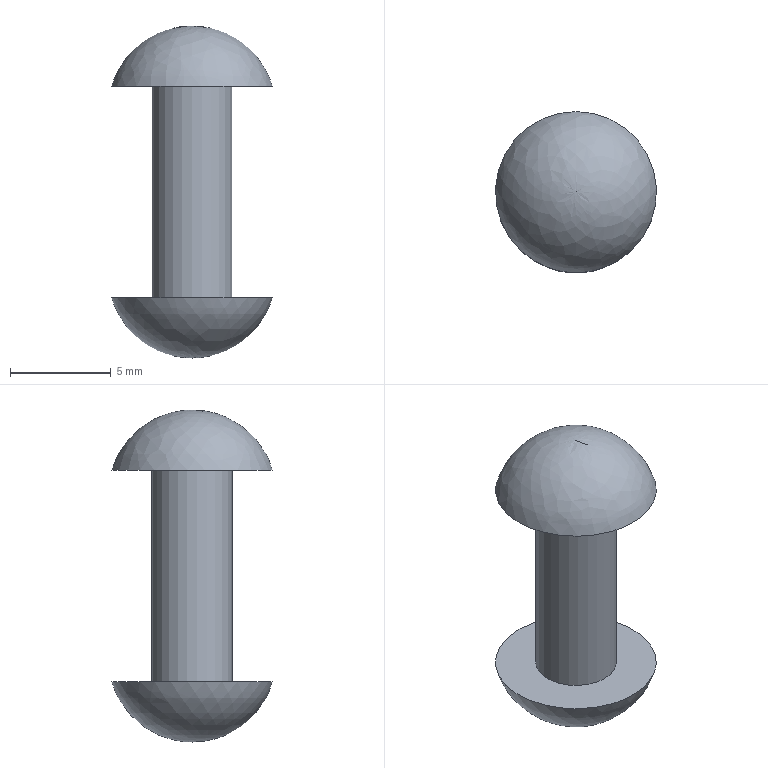Component | NX | RIVET4X13L | 1 solid | 5 faces | box 8 x 8 x 16.5 mm | volume 311 mm3 | spline 2 | plane 2 | cylinder 1 | commonest cylinder face diameters 4 x1
STEP:
#1=CARTESIAN_POINT('',(0.,0.,0.));
#2=DIRECTION('',(0.,0.,1.));
#3=DIRECTION('',(1.,0.,0.));
#4=AXIS2_PLACEMENT_3D('',#1,#2,#3);
#5=CARTESIAN_POINT('',(0.,84.,24.));
#6=VERTEX_POINT('',#5);
#7=CARTESIAN_POINT('',(0.,80.,27.));
#8=VERTEX_POINT('',#7);
#9=CARTESIAN_POINT('',(0.,84.,24.));
#10=CARTESIAN_POINT('',(0.,83.461,25.845));
#11=CARTESIAN_POINT('',(0.,81.923,26.999));
#12=CARTESIAN_POINT('',(0.,80.,27.));
#13=(BOUNDED_CURVE()B_SPLINE_CURVE(3,(#9,#10,#11,#12),.UNSPECIFIED.,.F.,.F.)B_SPLINE_CURVE_WITH_KNOTS((4,4),(0.,1.),.PIECEWISE_BEZIER_KNOTS.)CURVE()GEOMETRIC_REPRESENTATION_ITEM()RATIONAL_B_SPLINE_CURVE((1.,0.8669,0.8669,1.))REPRESENTATION_ITEM(''));
#14=CARTESIAN_POINT('',(0.,84.,24.));
#15=CARTESIAN_POINT('',(8.,84.,24.));
#16=CARTESIAN_POINT('',(8.,76.,24.));
#17=CARTESIAN_POINT('',(0.,76.,24.));
#18=CARTESIAN_POINT('',(-8.,76.,24.));
#19=CARTESIAN_POINT('',(-8.,84.,24.));
#20=CARTESIAN_POINT('',(0.,84.,24.));
#21=CARTESIAN_POINT('',(0.,83.461,25.845));
#22=CARTESIAN_POINT('',(6.921,83.461,25.845));
#23=CARTESIAN_POINT('',(6.921,76.539,25.845));
#24=CARTESIAN_POINT('',(0.,76.539,25.845));
#25=CARTESIAN_POINT('',(-6.921,76.539,25.845));
#26=CARTESIAN_POINT('',(-6.921,83.461,25.845));
#27=CARTESIAN_POINT('',(0.,83.461,25.845));
#28=CARTESIAN_POINT('',(0.,81.923,26.999));
#29=CARTESIAN_POINT('',(3.845,81.923,26.999));
#30=CARTESIAN_POINT('',(3.845,78.077,26.999));
#31=CARTESIAN_POINT('',(0.,78.077,26.999));
#32=CARTESIAN_POINT('',(-3.845,78.077,26.999));
#33=CARTESIAN_POINT('',(-3.845,81.923,26.999));
#34=CARTESIAN_POINT('',(0.,81.923,26.999));
#35=CARTESIAN_POINT('',(0.,80.,27.));
#36=CARTESIAN_POINT('',(0.,80.,27.));
#37=CARTESIAN_POINT('',(0.,80.,27.));
#38=CARTESIAN_POINT('',(0.,80.,27.));
#39=CARTESIAN_POINT('',(0.,80.,27.));
#40=CARTESIAN_POINT('',(0.,80.,27.));
#41=CARTESIAN_POINT('',(0.,80.,27.));
#42=(BOUNDED_SURFACE()B_SPLINE_SURFACE(3,3,((#14,#15,#16,#17,#18,#19,#20),(#21,#22,#23,#24,#25,#26,#27),(#28,#29,#30,#31,#32,#33,#34),(#35,#36,#37,#38,#39,#40,#41)),.UNSPECIFIED.,.F.,.T.,.F.)B_SPLINE_SURFACE_WITH_KNOTS((4,4),(1,3,3,3,1),(0.,1.),(-0.5,0.,0.5,1.,1.5),.UNSPECIFIED.)GEOMETRIC_REPRESENTATION_ITEM()RATIONAL_B_SPLINE_SURFACE(((1.,0.3333,0.3333,1.,0.3333,0.3333,1.),(0.8669,0.289,0.289,0.8669,0.289,0.289,0.8669),(0.8669,0.289,0.289,0.8669,0.289,0.289,0.8669),(1.,0.3333,0.3333,1.,0.3333,0.3333,1.)))REPRESENTATION_ITEM('')SURFACE());
#43=CARTESIAN_POINT('',(0.,1.));
#44=DIRECTION('',(1.,0.));
#45=VECTOR('',#44,1.);
#46=LINE('',#43,#45);
#47=(GEOMETRIC_REPRESENTATION_CONTEXT(2)PARAMETRIC_REPRESENTATION_CONTEXT()REPRESENTATION_CONTEXT('',''));
#48=DEFINITIONAL_REPRESENTATION('',(#46),#47);
#49=PCURVE('',#42,#48);
#50=CARTESIAN_POINT('',(0.,0.));
#51=DIRECTION('',(1.,0.));
#52=VECTOR('',#51,1.);
#53=LINE('',#50,#52);
#54=(GEOMETRIC_REPRESENTATION_CONTEXT(2)PARAMETRIC_REPRESENTATION_CONTEXT()REPRESENTATION_CONTEXT('',''));
#55=DEFINITIONAL_REPRESENTATION('',(#53),#54);
#56=PCURVE('',#42,#55);
#57=SEAM_CURVE('',#13,(#49,#56),.PCURVE_S1.);
#58=EDGE_CURVE('',#6,#8,#57,.T.);
#59=ORIENTED_EDGE('',*,*,#58,.F.);
#60=CARTESIAN_POINT('',(0.,80.,24.));
#61=DIRECTION('',(0.,0.,-1.));
#62=DIRECTION('',(0.,1.,0.));
#63=AXIS2_PLACEMENT_3D('',#60,#61,#62);
#64=CIRCLE('',#63,4.);
#65=CARTESIAN_POINT('',(0.,0.));
#66=CARTESIAN_POINT('',(0.,0.02352));
#67=CARTESIAN_POINT('',(0.,0.06491));
#68=CARTESIAN_POINT('',(0.,0.1146));
#69=CARTESIAN_POINT('',(0.,0.1575));
#70=CARTESIAN_POINT('',(0.,0.196));
#71=CARTESIAN_POINT('',(0.,0.2322));
#72=CARTESIAN_POINT('',(0.,0.2678));
#73=CARTESIAN_POINT('',(0.,0.304));
#74=CARTESIAN_POINT('',(0.,0.3425));
#75=CARTESIAN_POINT('',(0.,0.3856));
#76=CARTESIAN_POINT('',(0.,0.4343));
#77=CARTESIAN_POINT('',(0.,0.5));
#78=CARTESIAN_POINT('',(0.,0.5657));
#79=CARTESIAN_POINT('',(0.,0.6144));
#80=CARTESIAN_POINT('',(0.,0.6575));
#81=CARTESIAN_POINT('',(0.,0.696));
#82=CARTESIAN_POINT('',(0.,0.7322));
#83=CARTESIAN_POINT('',(0.,0.7678));
#84=CARTESIAN_POINT('',(0.,0.804));
#85=CARTESIAN_POINT('',(0.,0.8425));
#86=CARTESIAN_POINT('',(0.,0.8854));
#87=CARTESIAN_POINT('',(0.,0.9351));
#88=CARTESIAN_POINT('',(0.,0.9765));
#89=CARTESIAN_POINT('',(0.,1.));
#90=B_SPLINE_CURVE_WITH_KNOTS('',3,(#65,#66,#67,#68,#69,#70,#71,#72,#73,#74,#75,#76,#77,#78,#79,#80,#81,#82,#83,#84,#85,#86,#87,#88,#89),.UNSPECIFIED.,.F.,.F.,(4,1,1,1,1,1,1,1,1,1,1,1,1,1,1,1,1,1,1,1,1,1,4),(0.,0.2856,0.5712,0.8568,1.142,1.428,1.714,1.999,2.285,2.57,2.856,3.142,3.427,3.713,3.998,4.284,4.57,4.855,5.141,5.426,5.712,5.998,6.283),.QUASI_UNIFORM_KNOTS.);
#91=(GEOMETRIC_REPRESENTATION_CONTEXT(2)PARAMETRIC_REPRESENTATION_CONTEXT()REPRESENTATION_CONTEXT('',''));
#92=DEFINITIONAL_REPRESENTATION('',(#90),#91);
#93=PCURVE('',#42,#92);
#94=CARTESIAN_POINT('',(2.,80.,24.));
#95=DIRECTION('',(0.,0.,-1.));
#96=DIRECTION('',(0.,1.,0.));
#97=AXIS2_PLACEMENT_3D('',#94,#95,#96);
#98=PLANE('',#97);
#99=CARTESIAN_POINT('',(0.,-2.));
#100=DIRECTION('',(1.,0.));
#101=AXIS2_PLACEMENT_2D('',#99,#100);
#102=CIRCLE('',#101,4.);
#103=(GEOMETRIC_REPRESENTATION_CONTEXT(2)PARAMETRIC_REPRESENTATION_CONTEXT()REPRESENTATION_CONTEXT('',''));
#104=DEFINITIONAL_REPRESENTATION('',(#102),#103);
#105=PCURVE('',#98,#104);
#106=SURFACE_CURVE('',#64,(#93,#105),.PCURVE_S1.);
#107=EDGE_CURVE('',#6,#6,#106,.T.);
#108=ORIENTED_EDGE('',*,*,#107,.F.);
#109=ORIENTED_EDGE('',*,*,#58,.T.);
#110=EDGE_LOOP('',(#59,#108,#109));
#111=FACE_BOUND('',#110,.T.);
#112=ADVANCED_FACE('',(#111),#42,.T.);
#113=CARTESIAN_POINT('',(0.,84.,13.5));
#114=VERTEX_POINT('',#113);
#115=CARTESIAN_POINT('',(0.,80.,13.5));
#116=DIRECTION('',(0.,0.,-1.));
#117=DIRECTION('',(0.,1.,0.));
#118=AXIS2_PLACEMENT_3D('',#115,#116,#117);
#119=CIRCLE('',#118,4.);
#120=CARTESIAN_POINT('',(0.,80.,10.5));
#121=CARTESIAN_POINT('',(0.,80.,10.5));
#122=CARTESIAN_POINT('',(0.,80.,10.5));
#123=CARTESIAN_POINT('',(0.,80.,10.5));
#124=CARTESIAN_POINT('',(0.,80.,10.5));
#125=CARTESIAN_POINT('',(0.,80.,10.5));
#126=CARTESIAN_POINT('',(0.,80.,10.5));
#127=CARTESIAN_POINT('',(0.,81.923,10.501));
#128=CARTESIAN_POINT('',(3.845,81.923,10.501));
#129=CARTESIAN_POINT('',(3.845,78.077,10.501));
#130=CARTESIAN_POINT('',(0.,78.077,10.501));
#131=CARTESIAN_POINT('',(-3.845,78.077,10.501));
#132=CARTESIAN_POINT('',(-3.845,81.923,10.501));
#133=CARTESIAN_POINT('',(0.,81.923,10.501));
#134=CARTESIAN_POINT('',(0.,83.461,11.655));
#135=CARTESIAN_POINT('',(6.921,83.461,11.655));
#136=CARTESIAN_POINT('',(6.921,76.539,11.655));
#137=CARTESIAN_POINT('',(0.,76.539,11.655));
#138=CARTESIAN_POINT('',(-6.921,76.539,11.655));
#139=CARTESIAN_POINT('',(-6.921,83.461,11.655));
#140=CARTESIAN_POINT('',(0.,83.461,11.655));
#141=CARTESIAN_POINT('',(0.,84.,13.5));
#142=CARTESIAN_POINT('',(8.,84.,13.5));
#143=CARTESIAN_POINT('',(8.,76.,13.5));
#144=CARTESIAN_POINT('',(0.,76.,13.5));
#145=CARTESIAN_POINT('',(-8.,76.,13.5));
#146=CARTESIAN_POINT('',(-8.,84.,13.5));
#147=CARTESIAN_POINT('',(0.,84.,13.5));
#148=(BOUNDED_SURFACE()B_SPLINE_SURFACE(3,3,((#120,#121,#122,#123,#124,#125,#126),(#127,#128,#129,#130,#131,#132,#133),(#134,#135,#136,#137,#138,#139,#140),(#141,#142,#143,#144,#145,#146,#147)),.UNSPECIFIED.,.F.,.T.,.F.)B_SPLINE_SURFACE_WITH_KNOTS((4,4),(1,3,3,3,1),(0.,1.),(-0.5,0.,0.5,1.,1.5),.UNSPECIFIED.)GEOMETRIC_REPRESENTATION_ITEM()RATIONAL_B_SPLINE_SURFACE(((1.,0.3333,0.3333,1.,0.3333,0.3333,1.),(0.8669,0.289,0.289,0.8669,0.289,0.289,0.8669),(0.8669,0.289,0.289,0.8669,0.289,0.289,0.8669),(1.,0.3333,0.3333,1.,0.3333,0.3333,1.)))REPRESENTATION_ITEM('')SURFACE());
#149=CARTESIAN_POINT('',(1.,0.));
#150=CARTESIAN_POINT('',(1.,0.02352));
#151=CARTESIAN_POINT('',(1.,0.06491));
#152=CARTESIAN_POINT('',(1.,0.1146));
#153=CARTESIAN_POINT('',(1.,0.1575));
#154=CARTESIAN_POINT('',(1.,0.196));
#155=CARTESIAN_POINT('',(1.,0.2322));
#156=CARTESIAN_POINT('',(1.,0.2678));
#157=CARTESIAN_POINT('',(1.,0.304));
#158=CARTESIAN_POINT('',(1.,0.3425));
#159=CARTESIAN_POINT('',(1.,0.3856));
#160=CARTESIAN_POINT('',(1.,0.4343));
#161=CARTESIAN_POINT('',(1.,0.5));
#162=CARTESIAN_POINT('',(1.,0.5657));
#163=CARTESIAN_POINT('',(1.,0.6144));
#164=CARTESIAN_POINT('',(1.,0.6575));
#165=CARTESIAN_POINT('',(1.,0.696));
#166=CARTESIAN_POINT('',(1.,0.7322));
#167=CARTESIAN_POINT('',(1.,0.7678));
#168=CARTESIAN_POINT('',(1.,0.804));
#169=CARTESIAN_POINT('',(1.,0.8425));
#170=CARTESIAN_POINT('',(1.,0.8854));
#171=CARTESIAN_POINT('',(1.,0.9351));
#172=CARTESIAN_POINT('',(1.,0.9765));
#173=CARTESIAN_POINT('',(1.,1.));
#174=B_SPLINE_CURVE_WITH_KNOTS('',3,(#149,#150,#151,#152,#153,#154,#155,#156,#157,#158,#159,#160,#161,#162,#163,#164,#165,#166,#167,#168,#169,#170,#171,#172,#173),.UNSPECIFIED.,.F.,.F.,(4,1,1,1,1,1,1,1,1,1,1,1,1,1,1,1,1,1,1,1,1,1,4),(0.,0.2856,0.5712,0.8568,1.142,1.428,1.714,1.999,2.285,2.57,2.856,3.142,3.427,3.713,3.998,4.284,4.57,4.855,5.141,5.426,5.712,5.998,6.283),.QUASI_UNIFORM_KNOTS.);
#175=(GEOMETRIC_REPRESENTATION_CONTEXT(2)PARAMETRIC_REPRESENTATION_CONTEXT()REPRESENTATION_CONTEXT('',''));
#176=DEFINITIONAL_REPRESENTATION('',(#174),#175);
#177=PCURVE('',#148,#176);
#178=CARTESIAN_POINT('',(4.,80.,13.5));
#179=DIRECTION('',(0.,0.,1.));
#180=DIRECTION('',(0.,-1.,0.));
#181=AXIS2_PLACEMENT_3D('',#178,#179,#180);
#182=PLANE('',#181);
#183=CARTESIAN_POINT('',(-4.,-4.));
#184=CARTESIAN_POINT('',(-4.,2.928));
#185=CARTESIAN_POINT('',(2.,-0.5359));
#186=CARTESIAN_POINT('',(8.,-4.));
#187=CARTESIAN_POINT('',(2.,-7.464));
#188=CARTESIAN_POINT('',(-4.,-10.928));
#189=CARTESIAN_POINT('',(-4.,-4.));
#190=(BOUNDED_CURVE()B_SPLINE_CURVE(2,(#183,#184,#185,#186,#187,#188,#189),.UNSPECIFIED.,.T.,.F.)B_SPLINE_CURVE_WITH_KNOTS((1,2,2,2,2,1),(-2.094,0.,2.094,4.189,6.283,8.378),.UNSPECIFIED.)CURVE()GEOMETRIC_REPRESENTATION_ITEM()RATIONAL_B_SPLINE_CURVE((1.,0.5,1.,0.5,1.,0.5,1.))REPRESENTATION_ITEM(''));
#191=(GEOMETRIC_REPRESENTATION_CONTEXT(2)PARAMETRIC_REPRESENTATION_CONTEXT()REPRESENTATION_CONTEXT('',''));
#192=DEFINITIONAL_REPRESENTATION('',(#190),#191);
#193=PCURVE('',#182,#192);
#194=SURFACE_CURVE('',#119,(#177,#193),.PCURVE_S1.);
#195=EDGE_CURVE('',#114,#114,#194,.T.);
#196=ORIENTED_EDGE('',*,*,#195,.T.);
#197=CARTESIAN_POINT('',(0.,80.,10.5));
#198=VERTEX_POINT('',#197);
#199=CARTESIAN_POINT('',(0.,80.,10.5));
#200=CARTESIAN_POINT('',(0.,81.923,10.501));
#201=CARTESIAN_POINT('',(0.,83.461,11.655));
#202=CARTESIAN_POINT('',(0.,84.,13.5));
#203=(BOUNDED_CURVE()B_SPLINE_CURVE(3,(#199,#200,#201,#202),.UNSPECIFIED.,.F.,.F.)B_SPLINE_CURVE_WITH_KNOTS((4,4),(0.,1.),.PIECEWISE_BEZIER_KNOTS.)CURVE()GEOMETRIC_REPRESENTATION_ITEM()RATIONAL_B_SPLINE_CURVE((1.,0.8669,0.8669,1.))REPRESENTATION_ITEM(''));
#204=CARTESIAN_POINT('',(0.,1.));
#205=DIRECTION('',(1.,0.));
#206=VECTOR('',#205,1.);
#207=LINE('',#204,#206);
#208=(GEOMETRIC_REPRESENTATION_CONTEXT(2)PARAMETRIC_REPRESENTATION_CONTEXT()REPRESENTATION_CONTEXT('',''));
#209=DEFINITIONAL_REPRESENTATION('',(#207),#208);
#210=PCURVE('',#148,#209);
#211=CARTESIAN_POINT('',(0.,0.));
#212=DIRECTION('',(1.,0.));
#213=VECTOR('',#212,1.);
#214=LINE('',#211,#213);
#215=(GEOMETRIC_REPRESENTATION_CONTEXT(2)PARAMETRIC_REPRESENTATION_CONTEXT()REPRESENTATION_CONTEXT('',''));
#216=DEFINITIONAL_REPRESENTATION('',(#214),#215);
#217=PCURVE('',#148,#216);
#218=SEAM_CURVE('',#203,(#210,#217),.PCURVE_S1.);
#219=EDGE_CURVE('',#198,#114,#218,.T.);
#220=ORIENTED_EDGE('',*,*,#219,.F.);
#221=ORIENTED_EDGE('',*,*,#219,.T.);
#222=EDGE_LOOP('',(#196,#220,#221));
#223=FACE_BOUND('',#222,.T.);
#224=ADVANCED_FACE('',(#223),#148,.T.);
#225=CARTESIAN_POINT('',(0.,82.,13.5));
#226=VERTEX_POINT('',#225);
#227=CARTESIAN_POINT('',(0.,80.,13.5));
#228=DIRECTION('',(0.,0.,-1.));
#229=DIRECTION('',(0.,1.,0.));
#230=AXIS2_PLACEMENT_3D('',#227,#228,#229);
#231=CIRCLE('',#230,2.);
#232=CARTESIAN_POINT('',(-2.,-4.));
#233=CARTESIAN_POINT('',(-2.,-0.5359));
#234=CARTESIAN_POINT('',(1.,-2.268));
#235=CARTESIAN_POINT('',(4.,-4.));
#236=CARTESIAN_POINT('',(1.,-5.732));
#237=CARTESIAN_POINT('',(-2.,-7.464));
#238=CARTESIAN_POINT('',(-2.,-4.));
#239=(BOUNDED_CURVE()B_SPLINE_CURVE(2,(#232,#233,#234,#235,#236,#237,#238),.UNSPECIFIED.,.T.,.F.)B_SPLINE_CURVE_WITH_KNOTS((1,2,2,2,2,1),(-2.094,0.,2.094,4.189,6.283,8.378),.UNSPECIFIED.)CURVE()GEOMETRIC_REPRESENTATION_ITEM()RATIONAL_B_SPLINE_CURVE((1.,0.5,1.,0.5,1.,0.5,1.))REPRESENTATION_ITEM(''));
#240=(GEOMETRIC_REPRESENTATION_CONTEXT(2)PARAMETRIC_REPRESENTATION_CONTEXT()REPRESENTATION_CONTEXT('',''));
#241=DEFINITIONAL_REPRESENTATION('',(#239),#240);
#242=PCURVE('',#182,#241);
#243=CARTESIAN_POINT('',(0.,80.,10.5));
#244=DIRECTION('',(0.,0.,-1.));
#245=DIRECTION('',(0.,1.,0.));
#246=AXIS2_PLACEMENT_3D('',#243,#244,#245);
#247=CYLINDRICAL_SURFACE('',#246,2.);
#248=CARTESIAN_POINT('',(0.,-3.));
#249=DIRECTION('',(1.,0.));
#250=VECTOR('',#249,1.);
#251=LINE('',#248,#250);
#252=(GEOMETRIC_REPRESENTATION_CONTEXT(2)PARAMETRIC_REPRESENTATION_CONTEXT()REPRESENTATION_CONTEXT('',''));
#253=DEFINITIONAL_REPRESENTATION('',(#251),#252);
#254=PCURVE('',#247,#253);
#255=SURFACE_CURVE('',#231,(#242,#254),.PCURVE_S1.);
#256=EDGE_CURVE('',#226,#226,#255,.T.);
#257=ORIENTED_EDGE('',*,*,#256,.T.);
#258=EDGE_LOOP('',(#257));
#259=FACE_BOUND('',#258,.T.);
#260=ORIENTED_EDGE('',*,*,#195,.F.);
#261=EDGE_LOOP('',(#260));
#262=FACE_BOUND('',#261,.T.);
#263=ADVANCED_FACE('',(#259,#262),#182,.T.);
#264=CARTESIAN_POINT('',(0.,82.,24.));
#265=VERTEX_POINT('',#264);
#266=CARTESIAN_POINT('',(0.,80.,24.));
#267=DIRECTION('',(0.,0.,-1.));
#268=DIRECTION('',(0.,1.,0.));
#269=AXIS2_PLACEMENT_3D('',#266,#267,#268);
#270=CIRCLE('',#269,2.);
#271=CARTESIAN_POINT('',(0.,-13.5));
#272=DIRECTION('',(1.,0.));
#273=VECTOR('',#272,1.);
#274=LINE('',#271,#273);
#275=(GEOMETRIC_REPRESENTATION_CONTEXT(2)PARAMETRIC_REPRESENTATION_CONTEXT()REPRESENTATION_CONTEXT('',''));
#276=DEFINITIONAL_REPRESENTATION('',(#274),#275);
#277=PCURVE('',#247,#276);
#278=CARTESIAN_POINT('',(0.,-2.));
#279=DIRECTION('',(1.,0.));
#280=AXIS2_PLACEMENT_2D('',#278,#279);
#281=CIRCLE('',#280,2.);
#282=(GEOMETRIC_REPRESENTATION_CONTEXT(2)PARAMETRIC_REPRESENTATION_CONTEXT()REPRESENTATION_CONTEXT('',''));
#283=DEFINITIONAL_REPRESENTATION('',(#281),#282);
#284=PCURVE('',#98,#283);
#285=SURFACE_CURVE('',#270,(#277,#284),.PCURVE_S1.);
#286=EDGE_CURVE('',#265,#265,#285,.T.);
#287=ORIENTED_EDGE('',*,*,#286,.T.);
#288=CARTESIAN_POINT('',(0.,82.,24.));
#289=CARTESIAN_POINT('',(0.,82.,13.5));
#290=B_SPLINE_CURVE_WITH_KNOTS('',1,(#288,#289),.UNSPECIFIED.,.F.,.F.,(2,2),(-13.5,-3.),.PIECEWISE_BEZIER_KNOTS.);
#291=CARTESIAN_POINT('',(6.283,0.));
#292=DIRECTION('',(0.,1.));
#293=VECTOR('',#292,1.);
#294=LINE('',#291,#293);
#295=(GEOMETRIC_REPRESENTATION_CONTEXT(2)PARAMETRIC_REPRESENTATION_CONTEXT()REPRESENTATION_CONTEXT('',''));
#296=DEFINITIONAL_REPRESENTATION('',(#294),#295);
#297=PCURVE('',#247,#296);
#298=CARTESIAN_POINT('',(0.,0.));
#299=DIRECTION('',(0.,1.));
#300=VECTOR('',#299,1.);
#301=LINE('',#298,#300);
#302=(GEOMETRIC_REPRESENTATION_CONTEXT(2)PARAMETRIC_REPRESENTATION_CONTEXT()REPRESENTATION_CONTEXT('',''));
#303=DEFINITIONAL_REPRESENTATION('',(#301),#302);
#304=PCURVE('',#247,#303);
#305=SEAM_CURVE('',#290,(#297,#304),.PCURVE_S1.);
#306=EDGE_CURVE('',#265,#226,#305,.T.);
#307=ORIENTED_EDGE('',*,*,#306,.T.);
#308=ORIENTED_EDGE('',*,*,#256,.F.);
#309=ORIENTED_EDGE('',*,*,#306,.F.);
#310=EDGE_LOOP('',(#287,#307,#308,#309));
#311=FACE_BOUND('',#310,.T.);
#312=ADVANCED_FACE('',(#311),#247,.T.);
#313=ORIENTED_EDGE('',*,*,#107,.T.);
#314=EDGE_LOOP('',(#313));
#315=FACE_BOUND('',#314,.T.);
#316=ORIENTED_EDGE('',*,*,#286,.F.);
#317=EDGE_LOOP('',(#316));
#318=FACE_BOUND('',#317,.T.);
#319=ADVANCED_FACE('',(#315,#318),#98,.T.);
#320=CLOSED_SHELL('',(#112,#224,#263,#312,#319));
#321=MANIFOLD_SOLID_BREP('',#320);
#322=(LENGTH_UNIT()NAMED_UNIT(*)SI_UNIT(.MILLI.,.METRE.));
#323=UNCERTAINTY_MEASURE_WITH_UNIT(LENGTH_MEASURE(0.00001),#322,'','');
#324=(NAMED_UNIT(*)PLANE_ANGLE_UNIT()SI_UNIT($,.RADIAN.));
#325=(NAMED_UNIT(*)SI_UNIT($,.STERADIAN.)SOLID_ANGLE_UNIT());
#326=(GEOMETRIC_REPRESENTATION_CONTEXT(3)GLOBAL_UNCERTAINTY_ASSIGNED_CONTEXT((#323))GLOBAL_UNIT_ASSIGNED_CONTEXT((#322,#324,#325))REPRESENTATION_CONTEXT('',''));
#327=ADVANCED_BREP_SHAPE_REPRESENTATION('',(#4,#321),#326);